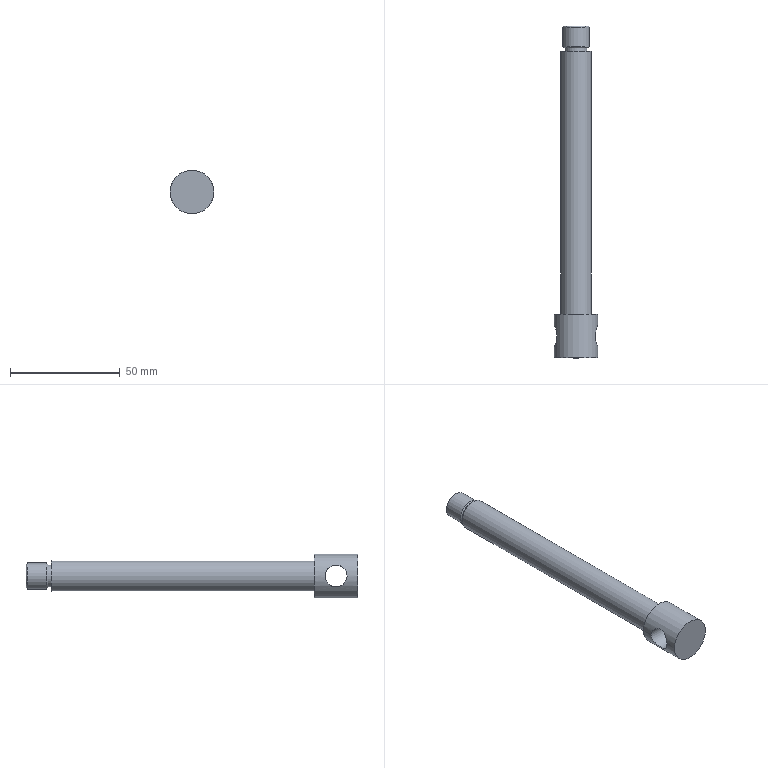Component | NX | SCREW_ROD | 1 solid | 12 faces | box 20 x 151.5 x 20 mm | volume 24476 mm3 | cylinder 5 | plane 5 | cone 2 | commonest cylinder face diameters 10 x2 20 x1 12 x1 14 x1
STEP:
#1=CARTESIAN_POINT('',(0.,0.,0.));
#2=DIRECTION('',(0.,0.,1.));
#3=DIRECTION('',(1.,0.,0.));
#4=AXIS2_PLACEMENT_3D('',#1,#2,#3);
#5=CARTESIAN_POINT('',(10.,-150.,-189.));
#6=VERTEX_POINT('',#5);
#7=CARTESIAN_POINT('',(0.,-150.,-189.));
#8=DIRECTION('',(0.,-1.,0.));
#9=DIRECTION('',(1.,0.,0.));
#10=AXIS2_PLACEMENT_3D('',#7,#8,#9);
#11=CIRCLE('',#10,10.);
#12=CARTESIAN_POINT('',(0.,-150.,-189.));
#13=DIRECTION('',(0.,1.,0.));
#14=DIRECTION('',(-1.,0.,0.));
#15=AXIS2_PLACEMENT_3D('',#12,#13,#14);
#16=CYLINDRICAL_SURFACE('',#15,10.);
#17=CARTESIAN_POINT('',(9.425,0.));
#18=DIRECTION('',(-1.,0.));
#19=VECTOR('',#18,1.);
#20=LINE('',#17,#19);
#21=(GEOMETRIC_REPRESENTATION_CONTEXT(2)PARAMETRIC_REPRESENTATION_CONTEXT()REPRESENTATION_CONTEXT('',''));
#22=DEFINITIONAL_REPRESENTATION('',(#20),#21);
#23=PCURVE('',#16,#22);
#24=CARTESIAN_POINT('',(0.,-150.,-189.));
#25=DIRECTION('',(0.,-1.,0.));
#26=DIRECTION('',(1.,0.,0.));
#27=AXIS2_PLACEMENT_3D('',#24,#25,#26);
#28=PLANE('',#27);
#29=CARTESIAN_POINT('',(0.,0.));
#30=DIRECTION('',(1.,0.));
#31=AXIS2_PLACEMENT_2D('',#29,#30);
#32=CIRCLE('',#31,10.);
#33=(GEOMETRIC_REPRESENTATION_CONTEXT(2)PARAMETRIC_REPRESENTATION_CONTEXT()REPRESENTATION_CONTEXT('',''));
#34=DEFINITIONAL_REPRESENTATION('',(#32),#33);
#35=PCURVE('',#28,#34);
#36=SURFACE_CURVE('',#11,(#23,#35),.PCURVE_S1.);
#37=EDGE_CURVE('',#6,#6,#36,.T.);
#38=ORIENTED_EDGE('',*,*,#37,.F.);
#39=CARTESIAN_POINT('',(10.,-145.,-189.));
#40=VERTEX_POINT('',#39);
#41=CARTESIAN_POINT('',(10.,-150.,-189.));
#42=CARTESIAN_POINT('',(10.,-145.,-189.));
#43=B_SPLINE_CURVE_WITH_KNOTS('',1,(#41,#42),.UNSPECIFIED.,.F.,.F.,(2,2),(0.,5.),.PIECEWISE_BEZIER_KNOTS.);
#44=CARTESIAN_POINT('',(9.425,0.));
#45=DIRECTION('',(0.,1.));
#46=VECTOR('',#45,1.);
#47=LINE('',#44,#46);
#48=(GEOMETRIC_REPRESENTATION_CONTEXT(2)PARAMETRIC_REPRESENTATION_CONTEXT()REPRESENTATION_CONTEXT('',''));
#49=DEFINITIONAL_REPRESENTATION('',(#47),#48);
#50=PCURVE('',#16,#49);
#51=CARTESIAN_POINT('',(3.142,0.));
#52=DIRECTION('',(0.,1.));
#53=VECTOR('',#52,1.);
#54=LINE('',#51,#53);
#55=(GEOMETRIC_REPRESENTATION_CONTEXT(2)PARAMETRIC_REPRESENTATION_CONTEXT()REPRESENTATION_CONTEXT('',''));
#56=DEFINITIONAL_REPRESENTATION('',(#54),#55);
#57=PCURVE('',#16,#56);
#58=SEAM_CURVE('',#43,(#50,#57),.PCURVE_S1.);
#59=EDGE_CURVE('',#6,#40,#58,.T.);
#60=ORIENTED_EDGE('',*,*,#59,.T.);
#61=CARTESIAN_POINT('',(10.,-135.,-189.));
#62=VERTEX_POINT('',#61);
#63=CARTESIAN_POINT('',(10.,-145.,-187.655));
#64=CARTESIAN_POINT('',(10.,-145.,-190.345));
#65=CARTESIAN_POINT('',(9.696,-144.44,-191.632));
#66=CARTESIAN_POINT('',(9.011,-142.627,-193.443));
#67=CARTESIAN_POINT('',(8.662,-141.341,-193.997));
#68=CARTESIAN_POINT('',(8.658,-138.682,-194.003));
#69=CARTESIAN_POINT('',(9.009,-137.38,-193.448));
#70=CARTESIAN_POINT('',(9.694,-135.563,-191.638));
#71=CARTESIAN_POINT('',(9.998,-135.004,-190.34));
#72=CARTESIAN_POINT('',(10.002,-134.996,-187.687));
#73=CARTESIAN_POINT('',(9.699,-135.553,-186.377));
#74=CARTESIAN_POINT('',(9.011,-137.371,-184.556));
#75=CARTESIAN_POINT('',(8.662,-138.664,-184.003));
#76=CARTESIAN_POINT('',(8.658,-141.312,-183.997));
#77=CARTESIAN_POINT('',(9.007,-142.615,-184.547));
#78=CARTESIAN_POINT('',(9.697,-144.445,-186.371));
#79=CARTESIAN_POINT('',(10.,-145.,-187.655));
#80=CARTESIAN_POINT('',(10.,-145.,-190.345));
#81=B_SPLINE_CURVE_WITH_KNOTS('',3,(#63,#64,#65,#66,#67,#68,#69,#70,#71,#72,#73,#74,#75,#76,#77,#78,#79,#80),.UNSPECIFIED.,.T.,.F.,(2,2,2,2,2,2,2,2,2,2,2),(-0.125,0.,0.125,0.25,0.375,0.5,0.625,0.75,0.875,1.,1.125),.UNSPECIFIED.);
#82=CARTESIAN_POINT('',(9.425,5.));
#83=CARTESIAN_POINT('',(9.449,5.));
#84=CARTESIAN_POINT('',(9.498,5.037));
#85=CARTESIAN_POINT('',(9.569,5.196));
#86=CARTESIAN_POINT('',(9.637,5.45));
#87=CARTESIAN_POINT('',(9.701,5.793));
#88=CARTESIAN_POINT('',(9.76,6.216));
#89=CARTESIAN_POINT('',(9.813,6.711));
#90=CARTESIAN_POINT('',(9.859,7.276));
#91=CARTESIAN_POINT('',(9.897,7.898));
#92=CARTESIAN_POINT('',(9.926,8.566));
#93=CARTESIAN_POINT('',(9.944,9.266));
#94=CARTESIAN_POINT('',(9.951,9.988));
#95=CARTESIAN_POINT('',(9.944,10.712));
#96=CARTESIAN_POINT('',(9.926,11.415));
#97=CARTESIAN_POINT('',(9.897,12.087));
#98=CARTESIAN_POINT('',(9.86,12.714));
#99=CARTESIAN_POINT('',(9.814,13.283));
#100=CARTESIAN_POINT('',(9.761,13.779));
#101=CARTESIAN_POINT('',(9.701,14.203));
#102=CARTESIAN_POINT('',(9.637,14.546));
#103=CARTESIAN_POINT('',(9.569,14.801));
#104=CARTESIAN_POINT('',(9.498,14.961));
#105=CARTESIAN_POINT('',(9.426,15.018));
#106=CARTESIAN_POINT('',(9.354,14.965));
#107=CARTESIAN_POINT('',(9.283,14.808));
#108=CARTESIAN_POINT('',(9.214,14.554));
#109=CARTESIAN_POINT('',(9.15,14.212));
#110=CARTESIAN_POINT('',(9.09,13.789));
#111=CARTESIAN_POINT('',(9.037,13.292));
#112=CARTESIAN_POINT('',(8.991,12.725));
#113=CARTESIAN_POINT('',(8.953,12.101));
#114=CARTESIAN_POINT('',(8.924,11.432));
#115=CARTESIAN_POINT('',(8.906,10.733));
#116=CARTESIAN_POINT('',(8.899,10.013));
#117=CARTESIAN_POINT('',(8.905,9.291));
#118=CARTESIAN_POINT('',(8.923,8.589));
#119=CARTESIAN_POINT('',(8.952,7.917));
#120=CARTESIAN_POINT('',(8.99,7.288));
#121=CARTESIAN_POINT('',(9.036,6.717));
#122=CARTESIAN_POINT('',(9.089,6.217));
#123=CARTESIAN_POINT('',(9.149,5.792));
#124=CARTESIAN_POINT('',(9.213,5.449));
#125=CARTESIAN_POINT('',(9.281,5.195));
#126=CARTESIAN_POINT('',(9.352,5.037));
#127=CARTESIAN_POINT('',(9.4,5.));
#128=CARTESIAN_POINT('',(9.425,5.));
#129=B_SPLINE_CURVE_WITH_KNOTS('',3,(#82,#83,#84,#85,#86,#87,#88,#89,#90,#91,#92,#93,#94,#95,#96,#97,#98,#99,#100,#101,#102,#103,#104,#105,#106,#107,#108,#109,#110,#111,#112,#113,#114,#115,#116,#117,#118,#119,#120,#121,#122,#123,#124,#125,#126,#127,#128),.UNSPECIFIED.,.T.,.F.,(4,1,1,1,1,1,1,1,1,1,1,1,1,1,1,1,1,1,1,1,1,1,1,1,1,1,1,1,1,1,1,1,1,1,1,1,1,1,1,1,1,1,1,1,4),(0.,0.02273,0.04545,0.06818,0.09091,0.1136,0.1364,0.1591,0.1818,0.2045,0.2273,0.25,0.2727,0.2955,0.3182,0.3409,0.3636,0.3864,0.4091,0.4318,0.4545,0.4773,0.5,0.5227,0.5455,0.5682,0.5909,0.6136,0.6364,0.6591,0.6818,0.7045,0.7273,0.75,0.7727,0.7955,0.8182,0.8409,0.8636,0.8864,0.9091,0.9318,0.9545,0.9773,1.),.QUASI_UNIFORM_KNOTS.);
#130=(GEOMETRIC_REPRESENTATION_CONTEXT(2)PARAMETRIC_REPRESENTATION_CONTEXT()REPRESENTATION_CONTEXT('',''));
#131=DEFINITIONAL_REPRESENTATION('',(#129),#130);
#132=PCURVE('',#16,#131);
#133=CARTESIAN_POINT('',(20.,-140.,-189.));
#134=DIRECTION('',(-1.,0.,0.));
#135=DIRECTION('',(0.,-1.,0.));
#136=AXIS2_PLACEMENT_3D('',#133,#134,#135);
#137=CYLINDRICAL_SURFACE('',#136,5.);
#138=CARTESIAN_POINT('',(3.142,10.));
#139=CARTESIAN_POINT('',(3.093,10.));
#140=CARTESIAN_POINT('',(2.997,10.02));
#141=CARTESIAN_POINT('',(2.853,10.101));
#142=CARTESIAN_POINT('',(2.709,10.223));
#143=CARTESIAN_POINT('',(2.566,10.377));
#144=CARTESIAN_POINT('',(2.425,10.553));
#145=CARTESIAN_POINT('',(2.285,10.742));
#146=CARTESIAN_POINT('',(2.144,10.926));
#147=CARTESIAN_POINT('',(2.002,11.091));
#148=CARTESIAN_POINT('',(1.859,11.225));
#149=CARTESIAN_POINT('',(1.716,11.316));
#150=CARTESIAN_POINT('',(1.572,11.351));
#151=CARTESIAN_POINT('',(1.428,11.317));
#152=CARTESIAN_POINT('',(1.284,11.226));
#153=CARTESIAN_POINT('',(1.141,11.092));
#154=CARTESIAN_POINT('',(0.9984,10.926));
#155=CARTESIAN_POINT('',(0.8566,10.742));
#156=CARTESIAN_POINT('',(0.716,10.552));
#157=CARTESIAN_POINT('',(0.5747,10.376));
#158=CARTESIAN_POINT('',(0.4326,10.222));
#159=CARTESIAN_POINT('',(0.2897,10.101));
#160=CARTESIAN_POINT('',(0.1458,10.02));
#161=CARTESIAN_POINT('',(0.04883,10.));
#162=CARTESIAN_POINT('',(0.,10.));
#163=B_SPLINE_CURVE_WITH_KNOTS('',3,(#138,#139,#140,#141,#142,#143,#144,#145,#146,#147,#148,#149,#150,#151,#152,#153,#154,#155,#156,#157,#158,#159,#160,#161,#162),.UNSPECIFIED.,.F.,.F.,(4,1,1,1,1,1,1,1,1,1,1,1,1,1,1,1,1,1,1,1,1,1,4),(0.5004,0.5231,0.5459,0.5686,0.5913,0.614,0.6367,0.6594,0.6821,0.7048,0.7275,0.7502,0.7729,0.7956,0.8183,0.841,0.8638,0.8865,0.9092,0.9319,0.9546,0.9773,1.),.QUASI_UNIFORM_KNOTS.);
#164=(GEOMETRIC_REPRESENTATION_CONTEXT(2)PARAMETRIC_REPRESENTATION_CONTEXT()REPRESENTATION_CONTEXT('',''));
#165=DEFINITIONAL_REPRESENTATION('',(#163),#164);
#166=PCURVE('',#137,#165);
#167=SURFACE_CURVE('',#81,(#132,#166),.PCURVE_S1.);
#168=EDGE_CURVE('',#62,#40,#167,.T.);
#169=ORIENTED_EDGE('',*,*,#168,.F.);
#170=CARTESIAN_POINT('',(10.,-130.,-189.));
#171=VERTEX_POINT('',#170);
#172=CARTESIAN_POINT('',(10.,-135.,-189.));
#173=CARTESIAN_POINT('',(10.,-130.,-189.));
#174=B_SPLINE_CURVE_WITH_KNOTS('',1,(#172,#173),.UNSPECIFIED.,.F.,.F.,(2,2),(15.,20.),.PIECEWISE_BEZIER_KNOTS.);
#175=CARTESIAN_POINT('',(9.425,0.));
#176=DIRECTION('',(0.,1.));
#177=VECTOR('',#176,1.);
#178=LINE('',#175,#177);
#179=(GEOMETRIC_REPRESENTATION_CONTEXT(2)PARAMETRIC_REPRESENTATION_CONTEXT()REPRESENTATION_CONTEXT('',''));
#180=DEFINITIONAL_REPRESENTATION('',(#178),#179);
#181=PCURVE('',#16,#180);
#182=CARTESIAN_POINT('',(3.142,0.));
#183=DIRECTION('',(0.,1.));
#184=VECTOR('',#183,1.);
#185=LINE('',#182,#184);
#186=(GEOMETRIC_REPRESENTATION_CONTEXT(2)PARAMETRIC_REPRESENTATION_CONTEXT()REPRESENTATION_CONTEXT('',''));
#187=DEFINITIONAL_REPRESENTATION('',(#185),#186);
#188=PCURVE('',#16,#187);
#189=SEAM_CURVE('',#174,(#181,#188),.PCURVE_S1.);
#190=EDGE_CURVE('',#62,#171,#189,.T.);
#191=ORIENTED_EDGE('',*,*,#190,.T.);
#192=CARTESIAN_POINT('',(0.,-130.,-189.));
#193=DIRECTION('',(0.,-1.,0.));
#194=DIRECTION('',(1.,0.,0.));
#195=AXIS2_PLACEMENT_3D('',#192,#193,#194);
#196=CIRCLE('',#195,10.);
#197=CARTESIAN_POINT('',(9.425,20.));
#198=DIRECTION('',(-1.,0.));
#199=VECTOR('',#198,1.);
#200=LINE('',#197,#199);
#201=(GEOMETRIC_REPRESENTATION_CONTEXT(2)PARAMETRIC_REPRESENTATION_CONTEXT()REPRESENTATION_CONTEXT('',''));
#202=DEFINITIONAL_REPRESENTATION('',(#200),#201);
#203=PCURVE('',#16,#202);
#204=CARTESIAN_POINT('',(0.,-130.,-189.));
#205=DIRECTION('',(0.,-1.,0.));
#206=DIRECTION('',(1.,0.,0.));
#207=AXIS2_PLACEMENT_3D('',#204,#205,#206);
#208=PLANE('',#207);
#209=CARTESIAN_POINT('',(0.,0.));
#210=DIRECTION('',(1.,0.));
#211=AXIS2_PLACEMENT_2D('',#209,#210);
#212=CIRCLE('',#211,10.);
#213=(GEOMETRIC_REPRESENTATION_CONTEXT(2)PARAMETRIC_REPRESENTATION_CONTEXT()REPRESENTATION_CONTEXT('',''));
#214=DEFINITIONAL_REPRESENTATION('',(#212),#213);
#215=PCURVE('',#208,#214);
#216=SURFACE_CURVE('',#196,(#203,#215),.PCURVE_S1.);
#217=EDGE_CURVE('',#171,#171,#216,.T.);
#218=ORIENTED_EDGE('',*,*,#217,.T.);
#219=ORIENTED_EDGE('',*,*,#190,.F.);
#220=CARTESIAN_POINT('',(10.,-145.,-187.655));
#221=CARTESIAN_POINT('',(10.,-145.,-190.345));
#222=CARTESIAN_POINT('',(9.696,-144.44,-191.632));
#223=CARTESIAN_POINT('',(9.011,-142.627,-193.443));
#224=CARTESIAN_POINT('',(8.662,-141.341,-193.997));
#225=CARTESIAN_POINT('',(8.658,-138.682,-194.003));
#226=CARTESIAN_POINT('',(9.009,-137.38,-193.448));
#227=CARTESIAN_POINT('',(9.694,-135.563,-191.638));
#228=CARTESIAN_POINT('',(9.998,-135.004,-190.34));
#229=CARTESIAN_POINT('',(10.002,-134.996,-187.687));
#230=CARTESIAN_POINT('',(9.699,-135.553,-186.377));
#231=CARTESIAN_POINT('',(9.011,-137.371,-184.556));
#232=CARTESIAN_POINT('',(8.662,-138.664,-184.003));
#233=CARTESIAN_POINT('',(8.658,-141.312,-183.997));
#234=CARTESIAN_POINT('',(9.007,-142.615,-184.547));
#235=CARTESIAN_POINT('',(9.697,-144.445,-186.371));
#236=CARTESIAN_POINT('',(10.,-145.,-187.655));
#237=CARTESIAN_POINT('',(10.,-145.,-190.345));
#238=B_SPLINE_CURVE_WITH_KNOTS('',3,(#220,#221,#222,#223,#224,#225,#226,#227,#228,#229,#230,#231,#232,#233,#234,#235,#236,#237),.UNSPECIFIED.,.T.,.F.,(2,2,2,2,2,2,2,2,2,2,2),(-0.125,0.,0.125,0.25,0.375,0.5,0.625,0.75,0.875,1.,1.125),.UNSPECIFIED.);
#239=CARTESIAN_POINT('',(3.142,5.));
#240=CARTESIAN_POINT('',(3.166,5.));
#241=CARTESIAN_POINT('',(3.215,5.037));
#242=CARTESIAN_POINT('',(3.285,5.196));
#243=CARTESIAN_POINT('',(3.354,5.45));
#244=CARTESIAN_POINT('',(3.418,5.793));
#245=CARTESIAN_POINT('',(3.477,6.216));
#246=CARTESIAN_POINT('',(3.53,6.711));
#247=CARTESIAN_POINT('',(3.576,7.276));
#248=CARTESIAN_POINT('',(3.614,7.898));
#249=CARTESIAN_POINT('',(3.642,8.566));
#250=CARTESIAN_POINT('',(3.661,9.266));
#251=CARTESIAN_POINT('',(3.667,9.988));
#252=CARTESIAN_POINT('',(3.661,10.712));
#253=CARTESIAN_POINT('',(3.643,11.415));
#254=CARTESIAN_POINT('',(3.614,12.087));
#255=CARTESIAN_POINT('',(3.576,12.714));
#256=CARTESIAN_POINT('',(3.53,13.283));
#257=CARTESIAN_POINT('',(3.478,13.779));
#258=CARTESIAN_POINT('',(3.418,14.203));
#259=CARTESIAN_POINT('',(3.354,14.546));
#260=CARTESIAN_POINT('',(3.286,14.801));
#261=CARTESIAN_POINT('',(3.215,14.961));
#262=CARTESIAN_POINT('',(3.143,15.018));
#263=CARTESIAN_POINT('',(3.071,14.965));
#264=CARTESIAN_POINT('',(3.,14.808));
#265=CARTESIAN_POINT('',(2.931,14.554));
#266=CARTESIAN_POINT('',(2.866,14.212));
#267=CARTESIAN_POINT('',(2.807,13.789));
#268=CARTESIAN_POINT('',(2.754,13.292));
#269=CARTESIAN_POINT('',(2.707,12.725));
#270=CARTESIAN_POINT('',(2.67,12.101));
#271=CARTESIAN_POINT('',(2.641,11.432));
#272=CARTESIAN_POINT('',(2.622,10.733));
#273=CARTESIAN_POINT('',(2.616,10.013));
#274=CARTESIAN_POINT('',(2.622,9.291));
#275=CARTESIAN_POINT('',(2.64,8.589));
#276=CARTESIAN_POINT('',(2.669,7.917));
#277=CARTESIAN_POINT('',(2.707,7.288));
#278=CARTESIAN_POINT('',(2.753,6.717));
#279=CARTESIAN_POINT('',(2.806,6.217));
#280=CARTESIAN_POINT('',(2.865,5.792));
#281=CARTESIAN_POINT('',(2.93,5.449));
#282=CARTESIAN_POINT('',(2.998,5.195));
#283=CARTESIAN_POINT('',(3.069,5.037));
#284=CARTESIAN_POINT('',(3.117,5.));
#285=CARTESIAN_POINT('',(3.142,5.));
#286=B_SPLINE_CURVE_WITH_KNOTS('',3,(#239,#240,#241,#242,#243,#244,#245,#246,#247,#248,#249,#250,#251,#252,#253,#254,#255,#256,#257,#258,#259,#260,#261,#262,#263,#264,#265,#266,#267,#268,#269,#270,#271,#272,#273,#274,#275,#276,#277,#278,#279,#280,#281,#282,#283,#284,#285),.UNSPECIFIED.,.T.,.F.,(4,1,1,1,1,1,1,1,1,1,1,1,1,1,1,1,1,1,1,1,1,1,1,1,1,1,1,1,1,1,1,1,1,1,1,1,1,1,1,1,1,1,1,1,4),(0.,0.02273,0.04545,0.06818,0.09091,0.1136,0.1364,0.1591,0.1818,0.2045,0.2273,0.25,0.2727,0.2955,0.3182,0.3409,0.3636,0.3864,0.4091,0.4318,0.4545,0.4773,0.5,0.5227,0.5455,0.5682,0.5909,0.6136,0.6364,0.6591,0.6818,0.7045,0.7273,0.75,0.7727,0.7955,0.8182,0.8409,0.8636,0.8864,0.9091,0.9318,0.9545,0.9773,1.),.QUASI_UNIFORM_KNOTS.);
#287=(GEOMETRIC_REPRESENTATION_CONTEXT(2)PARAMETRIC_REPRESENTATION_CONTEXT()REPRESENTATION_CONTEXT('',''));
#288=DEFINITIONAL_REPRESENTATION('',(#286),#287);
#289=PCURVE('',#16,#288);
#290=CARTESIAN_POINT('',(6.283,10.));
#291=CARTESIAN_POINT('',(6.234,10.));
#292=CARTESIAN_POINT('',(6.137,10.02));
#293=CARTESIAN_POINT('',(5.993,10.101));
#294=CARTESIAN_POINT('',(5.85,10.223));
#295=CARTESIAN_POINT('',(5.708,10.377));
#296=CARTESIAN_POINT('',(5.567,10.553));
#297=CARTESIAN_POINT('',(5.427,10.742));
#298=CARTESIAN_POINT('',(5.286,10.925));
#299=CARTESIAN_POINT('',(5.144,11.09));
#300=CARTESIAN_POINT('',(5.001,11.225));
#301=CARTESIAN_POINT('',(4.858,11.316));
#302=CARTESIAN_POINT('',(4.713,11.351));
#303=CARTESIAN_POINT('',(4.568,11.317));
#304=CARTESIAN_POINT('',(4.424,11.225));
#305=CARTESIAN_POINT('',(4.281,11.09));
#306=CARTESIAN_POINT('',(4.138,10.924));
#307=CARTESIAN_POINT('',(3.997,10.74));
#308=CARTESIAN_POINT('',(3.857,10.551));
#309=CARTESIAN_POINT('',(3.716,10.376));
#310=CARTESIAN_POINT('',(3.573,10.222));
#311=CARTESIAN_POINT('',(3.43,10.101));
#312=CARTESIAN_POINT('',(3.286,10.02));
#313=CARTESIAN_POINT('',(3.19,10.));
#314=CARTESIAN_POINT('',(3.142,10.));
#315=B_SPLINE_CURVE_WITH_KNOTS('',3,(#290,#291,#292,#293,#294,#295,#296,#297,#298,#299,#300,#301,#302,#303,#304,#305,#306,#307,#308,#309,#310,#311,#312,#313,#314),.UNSPECIFIED.,.F.,.F.,(4,1,1,1,1,1,1,1,1,1,1,1,1,1,1,1,1,1,1,1,1,1,4),(0.,0.02275,0.04549,0.06824,0.09099,0.1137,0.1365,0.1592,0.182,0.2047,0.2275,0.2502,0.273,0.2957,0.3185,0.3412,0.364,0.3867,0.4094,0.4322,0.4549,0.4777,0.5004),.QUASI_UNIFORM_KNOTS.);
#316=(GEOMETRIC_REPRESENTATION_CONTEXT(2)PARAMETRIC_REPRESENTATION_CONTEXT()REPRESENTATION_CONTEXT('',''));
#317=DEFINITIONAL_REPRESENTATION('',(#315),#316);
#318=PCURVE('',#137,#317);
#319=SURFACE_CURVE('',#238,(#289,#318),.PCURVE_S1.);
#320=EDGE_CURVE('',#40,#62,#319,.T.);
#321=ORIENTED_EDGE('',*,*,#320,.F.);
#322=ORIENTED_EDGE('',*,*,#59,.F.);
#323=EDGE_LOOP('',(#38,#60,#169,#191,#218,#219,#321,#322));
#324=FACE_BOUND('',#323,.T.);
#325=CARTESIAN_POINT('',(-10.,-145.,-189.));
#326=VERTEX_POINT('',#325);
#327=CARTESIAN_POINT('',(-10.,-145.,-190.345));
#328=CARTESIAN_POINT('',(-10.,-145.,-187.655));
#329=CARTESIAN_POINT('',(-9.696,-144.44,-186.368));
#330=CARTESIAN_POINT('',(-9.011,-142.627,-184.557));
#331=CARTESIAN_POINT('',(-8.662,-141.341,-184.003));
#332=CARTESIAN_POINT('',(-8.658,-138.682,-183.997));
#333=CARTESIAN_POINT('',(-9.009,-137.38,-184.552));
#334=CARTESIAN_POINT('',(-9.694,-135.563,-186.362));
#335=CARTESIAN_POINT('',(-9.998,-135.004,-187.66));
#336=CARTESIAN_POINT('',(-10.002,-134.996,-190.313));
#337=CARTESIAN_POINT('',(-9.699,-135.553,-191.623));
#338=CARTESIAN_POINT('',(-9.011,-137.371,-193.444));
#339=CARTESIAN_POINT('',(-8.662,-138.664,-193.997));
#340=CARTESIAN_POINT('',(-8.658,-141.312,-194.003));
#341=CARTESIAN_POINT('',(-9.007,-142.615,-193.453));
#342=CARTESIAN_POINT('',(-9.697,-144.445,-191.629));
#343=CARTESIAN_POINT('',(-10.,-145.,-190.345));
#344=CARTESIAN_POINT('',(-10.,-145.,-187.655));
#345=B_SPLINE_CURVE_WITH_KNOTS('',3,(#327,#328,#329,#330,#331,#332,#333,#334,#335,#336,#337,#338,#339,#340,#341,#342,#343,#344),.UNSPECIFIED.,.T.,.F.,(2,2,2,2,2,2,2,2,2,2,2),(-0.125,0.,0.125,0.25,0.375,0.5,0.625,0.75,0.875,1.,1.125),.UNSPECIFIED.);
#346=CARTESIAN_POINT('',(6.283,5.));
#347=CARTESIAN_POINT('',(6.308,5.));
#348=CARTESIAN_POINT('',(6.356,5.037));
#349=CARTESIAN_POINT('',(6.427,5.196));
#350=CARTESIAN_POINT('',(6.495,5.45));
#351=CARTESIAN_POINT('',(6.559,5.793));
#352=CARTESIAN_POINT('',(6.619,6.216));
#353=CARTESIAN_POINT('',(6.671,6.711));
#354=CARTESIAN_POINT('',(6.717,7.276));
#355=CARTESIAN_POINT('',(6.755,7.898));
#356=CARTESIAN_POINT('',(6.784,8.566));
#357=CARTESIAN_POINT('',(6.802,9.266));
#358=CARTESIAN_POINT('',(6.809,9.988));
#359=CARTESIAN_POINT('',(6.803,10.712));
#360=CARTESIAN_POINT('',(6.784,11.415));
#361=CARTESIAN_POINT('',(6.756,12.087));
#362=CARTESIAN_POINT('',(6.718,12.714));
#363=CARTESIAN_POINT('',(6.672,13.283));
#364=CARTESIAN_POINT('',(6.619,13.779));
#365=CARTESIAN_POINT('',(6.56,14.203));
#366=CARTESIAN_POINT('',(6.496,14.546));
#367=CARTESIAN_POINT('',(6.427,14.801));
#368=CARTESIAN_POINT('',(6.357,14.961));
#369=CARTESIAN_POINT('',(6.285,15.018));
#370=CARTESIAN_POINT('',(6.212,14.965));
#371=CARTESIAN_POINT('',(6.141,14.808));
#372=CARTESIAN_POINT('',(6.073,14.554));
#373=CARTESIAN_POINT('',(6.008,14.212));
#374=CARTESIAN_POINT('',(5.948,13.789));
#375=CARTESIAN_POINT('',(5.895,13.292));
#376=CARTESIAN_POINT('',(5.849,12.725));
#377=CARTESIAN_POINT('',(5.811,12.101));
#378=CARTESIAN_POINT('',(5.782,11.432));
#379=CARTESIAN_POINT('',(5.764,10.733));
#380=CARTESIAN_POINT('',(5.757,10.013));
#381=CARTESIAN_POINT('',(5.764,9.291));
#382=CARTESIAN_POINT('',(5.782,8.589));
#383=CARTESIAN_POINT('',(5.81,7.917));
#384=CARTESIAN_POINT('',(5.848,7.288));
#385=CARTESIAN_POINT('',(5.894,6.717));
#386=CARTESIAN_POINT('',(5.948,6.217));
#387=CARTESIAN_POINT('',(6.007,5.792));
#388=CARTESIAN_POINT('',(6.071,5.449));
#389=CARTESIAN_POINT('',(6.139,5.195));
#390=CARTESIAN_POINT('',(6.21,5.037));
#391=CARTESIAN_POINT('',(6.259,5.));
#392=CARTESIAN_POINT('',(6.283,5.));
#393=B_SPLINE_CURVE_WITH_KNOTS('',3,(#346,#347,#348,#349,#350,#351,#352,#353,#354,#355,#356,#357,#358,#359,#360,#361,#362,#363,#364,#365,#366,#367,#368,#369,#370,#371,#372,#373,#374,#375,#376,#377,#378,#379,#380,#381,#382,#383,#384,#385,#386,#387,#388,#389,#390,#391,#392),.UNSPECIFIED.,.T.,.F.,(4,1,1,1,1,1,1,1,1,1,1,1,1,1,1,1,1,1,1,1,1,1,1,1,1,1,1,1,1,1,1,1,1,1,1,1,1,1,1,1,1,1,1,1,4),(0.,0.02273,0.04545,0.06818,0.09091,0.1136,0.1364,0.1591,0.1818,0.2045,0.2273,0.25,0.2727,0.2955,0.3182,0.3409,0.3636,0.3864,0.4091,0.4318,0.4545,0.4773,0.5,0.5227,0.5455,0.5682,0.5909,0.6136,0.6364,0.6591,0.6818,0.7045,0.7273,0.75,0.7727,0.7955,0.8182,0.8409,0.8636,0.8864,0.9091,0.9318,0.9545,0.9773,1.),.QUASI_UNIFORM_KNOTS.);
#394=(GEOMETRIC_REPRESENTATION_CONTEXT(2)PARAMETRIC_REPRESENTATION_CONTEXT()REPRESENTATION_CONTEXT('',''));
#395=DEFINITIONAL_REPRESENTATION('',(#393),#394);
#396=PCURVE('',#16,#395);
#397=CARTESIAN_POINT('',(0.,30.));
#398=CARTESIAN_POINT('',(0.04886,30.));
#399=CARTESIAN_POINT('',(0.146,29.98));
#400=CARTESIAN_POINT('',(0.2901,29.899));
#401=CARTESIAN_POINT('',(0.4332,29.777));
#402=CARTESIAN_POINT('',(0.5752,29.623));
#403=CARTESIAN_POINT('',(0.7161,29.448));
#404=CARTESIAN_POINT('',(0.8557,29.259));
#405=CARTESIAN_POINT('',(0.9964,29.076));
#406=CARTESIAN_POINT('',(1.138,28.911));
#407=CARTESIAN_POINT('',(1.281,28.776));
#408=CARTESIAN_POINT('',(1.424,28.684));
#409=CARTESIAN_POINT('',(1.568,28.649));
#410=CARTESIAN_POINT('',(1.713,28.683));
#411=CARTESIAN_POINT('',(1.857,28.773));
#412=CARTESIAN_POINT('',(2.,28.908));
#413=CARTESIAN_POINT('',(2.143,29.074));
#414=CARTESIAN_POINT('',(2.284,29.257));
#415=CARTESIAN_POINT('',(2.424,29.446));
#416=CARTESIAN_POINT('',(2.565,29.621));
#417=CARTESIAN_POINT('',(2.708,29.775));
#418=CARTESIAN_POINT('',(2.851,29.898));
#419=CARTESIAN_POINT('',(2.994,29.979));
#420=CARTESIAN_POINT('',(3.139,30.01));
#421=CARTESIAN_POINT('',(3.283,29.981));
#422=CARTESIAN_POINT('',(3.428,29.901));
#423=CARTESIAN_POINT('',(3.571,29.779));
#424=CARTESIAN_POINT('',(3.714,29.626));
#425=CARTESIAN_POINT('',(3.856,29.45));
#426=CARTESIAN_POINT('',(3.996,29.26));
#427=CARTESIAN_POINT('',(4.138,29.077));
#428=CARTESIAN_POINT('',(4.28,28.911));
#429=CARTESIAN_POINT('',(4.423,28.776));
#430=CARTESIAN_POINT('',(4.566,28.684));
#431=CARTESIAN_POINT('',(4.71,28.649));
#432=CARTESIAN_POINT('',(4.854,28.682));
#433=CARTESIAN_POINT('',(4.998,28.773));
#434=CARTESIAN_POINT('',(5.141,28.907));
#435=CARTESIAN_POINT('',(5.284,29.073));
#436=CARTESIAN_POINT('',(5.426,29.257));
#437=CARTESIAN_POINT('',(5.567,29.447));
#438=CARTESIAN_POINT('',(5.708,29.623));
#439=CARTESIAN_POINT('',(5.85,29.777));
#440=CARTESIAN_POINT('',(5.993,29.899));
#441=CARTESIAN_POINT('',(6.137,29.98));
#442=CARTESIAN_POINT('',(6.234,30.));
#443=CARTESIAN_POINT('',(6.283,30.));
#444=B_SPLINE_CURVE_WITH_KNOTS('',3,(#397,#398,#399,#400,#401,#402,#403,#404,#405,#406,#407,#408,#409,#410,#411,#412,#413,#414,#415,#416,#417,#418,#419,#420,#421,#422,#423,#424,#425,#426,#427,#428,#429,#430,#431,#432,#433,#434,#435,#436,#437,#438,#439,#440,#441,#442,#443),.UNSPECIFIED.,.F.,.F.,(4,1,1,1,1,1,1,1,1,1,1,1,1,1,1,1,1,1,1,1,1,1,1,1,1,1,1,1,1,1,1,1,1,1,1,1,1,1,1,1,1,1,1,1,4),(0.,0.02273,0.04545,0.06818,0.09091,0.1136,0.1364,0.1591,0.1818,0.2045,0.2273,0.25,0.2727,0.2955,0.3182,0.3409,0.3636,0.3864,0.4091,0.4318,0.4545,0.4773,0.5,0.5227,0.5455,0.5682,0.5909,0.6136,0.6364,0.6591,0.6818,0.7045,0.7273,0.75,0.7727,0.7955,0.8182,0.8409,0.8636,0.8864,0.9091,0.9318,0.9545,0.9773,1.),.QUASI_UNIFORM_KNOTS.);
#445=(GEOMETRIC_REPRESENTATION_CONTEXT(2)PARAMETRIC_REPRESENTATION_CONTEXT()REPRESENTATION_CONTEXT('',''));
#446=DEFINITIONAL_REPRESENTATION('',(#444),#445);
#447=PCURVE('',#137,#446);
#448=SURFACE_CURVE('',#345,(#396,#447),.PCURVE_S1.);
#449=EDGE_CURVE('',#326,#326,#448,.T.);
#450=ORIENTED_EDGE('',*,*,#449,.F.);
#451=EDGE_LOOP('',(#450));
#452=FACE_BOUND('',#451,.T.);
#453=ADVANCED_FACE('',(#324,#452),#16,.T.);
#454=CARTESIAN_POINT('',(6.,1.,-189.));
#455=VERTEX_POINT('',#454);
#456=CARTESIAN_POINT('',(0.,1.,-189.));
#457=DIRECTION('',(0.,-1.,0.));
#458=DIRECTION('',(1.,0.,0.));
#459=AXIS2_PLACEMENT_3D('',#456,#457,#458);
#460=CIRCLE('',#459,6.);
#461=CARTESIAN_POINT('',(0.,-8.5,-189.));
#462=DIRECTION('',(0.,1.,0.));
#463=DIRECTION('',(-1.,0.,0.));
#464=AXIS2_PLACEMENT_3D('',#461,#462,#463);
#465=CYLINDRICAL_SURFACE('',#464,6.);
#466=CARTESIAN_POINT('',(9.425,9.5));
#467=DIRECTION('',(-1.,0.));
#468=VECTOR('',#467,1.);
#469=LINE('',#466,#468);
#470=(GEOMETRIC_REPRESENTATION_CONTEXT(2)PARAMETRIC_REPRESENTATION_CONTEXT()REPRESENTATION_CONTEXT('',''));
#471=DEFINITIONAL_REPRESENTATION('',(#469),#470);
#472=PCURVE('',#465,#471);
#473=CARTESIAN_POINT('',(0.,1.,-189.));
#474=DIRECTION('',(0.,-1.,0.));
#475=DIRECTION('',(1.,0.,0.));
#476=AXIS2_PLACEMENT_3D('',#473,#474,#475);
#477=CONICAL_SURFACE('',#476,6.,0.7854);
#478=CARTESIAN_POINT('',(0.,0.));
#479=DIRECTION('',(1.,0.));
#480=VECTOR('',#479,1.);
#481=LINE('',#478,#480);
#482=(GEOMETRIC_REPRESENTATION_CONTEXT(2)PARAMETRIC_REPRESENTATION_CONTEXT()REPRESENTATION_CONTEXT('',''));
#483=DEFINITIONAL_REPRESENTATION('',(#481),#482);
#484=PCURVE('',#477,#483);
#485=SURFACE_CURVE('',#460,(#472,#484),.PCURVE_S1.);
#486=EDGE_CURVE('',#455,#455,#485,.T.);
#487=ORIENTED_EDGE('',*,*,#486,.T.);
#488=CARTESIAN_POINT('',(6.,-8.,-189.));
#489=VERTEX_POINT('',#488);
#490=CARTESIAN_POINT('',(6.,-8.,-189.));
#491=CARTESIAN_POINT('',(6.,1.,-189.));
#492=B_SPLINE_CURVE_WITH_KNOTS('',1,(#490,#491),.UNSPECIFIED.,.F.,.F.,(2,2),(0.5,9.5),.PIECEWISE_BEZIER_KNOTS.);
#493=CARTESIAN_POINT('',(3.142,0.));
#494=DIRECTION('',(0.,1.));
#495=VECTOR('',#494,1.);
#496=LINE('',#493,#495);
#497=(GEOMETRIC_REPRESENTATION_CONTEXT(2)PARAMETRIC_REPRESENTATION_CONTEXT()REPRESENTATION_CONTEXT('',''));
#498=DEFINITIONAL_REPRESENTATION('',(#496),#497);
#499=PCURVE('',#465,#498);
#500=CARTESIAN_POINT('',(9.425,0.));
#501=DIRECTION('',(0.,1.));
#502=VECTOR('',#501,1.);
#503=LINE('',#500,#502);
#504=(GEOMETRIC_REPRESENTATION_CONTEXT(2)PARAMETRIC_REPRESENTATION_CONTEXT()REPRESENTATION_CONTEXT('',''));
#505=DEFINITIONAL_REPRESENTATION('',(#503),#504);
#506=PCURVE('',#465,#505);
#507=SEAM_CURVE('',#492,(#499,#506),.PCURVE_S1.);
#508=EDGE_CURVE('',#489,#455,#507,.T.);
#509=ORIENTED_EDGE('',*,*,#508,.F.);
#510=CARTESIAN_POINT('',(0.,-8.,-189.));
#511=DIRECTION('',(0.,1.,0.));
#512=DIRECTION('',(1.,0.,0.));
#513=AXIS2_PLACEMENT_3D('',#510,#511,#512);
#514=CIRCLE('',#513,6.);
#515=CARTESIAN_POINT('',(3.142,0.5));
#516=DIRECTION('',(1.,0.));
#517=VECTOR('',#516,1.);
#518=LINE('',#515,#517);
#519=(GEOMETRIC_REPRESENTATION_CONTEXT(2)PARAMETRIC_REPRESENTATION_CONTEXT()REPRESENTATION_CONTEXT('',''));
#520=DEFINITIONAL_REPRESENTATION('',(#518),#519);
#521=PCURVE('',#465,#520);
#522=CARTESIAN_POINT('',(0.,-8.5,-189.));
#523=DIRECTION('',(0.,1.,0.));
#524=DIRECTION('',(-1.,0.,0.));
#525=AXIS2_PLACEMENT_3D('',#522,#523,#524);
#526=CONICAL_SURFACE('',#525,5.5,0.7854);
#527=CARTESIAN_POINT('',(3.142,0.5));
#528=DIRECTION('',(1.,0.));
#529=VECTOR('',#528,1.);
#530=LINE('',#527,#529);
#531=(GEOMETRIC_REPRESENTATION_CONTEXT(2)PARAMETRIC_REPRESENTATION_CONTEXT()REPRESENTATION_CONTEXT('',''));
#532=DEFINITIONAL_REPRESENTATION('',(#530),#531);
#533=PCURVE('',#526,#532);
#534=SURFACE_CURVE('',#514,(#521,#533),.PCURVE_S1.);
#535=EDGE_CURVE('',#489,#489,#534,.T.);
#536=ORIENTED_EDGE('',*,*,#535,.T.);
#537=ORIENTED_EDGE('',*,*,#508,.T.);
#538=EDGE_LOOP('',(#487,#509,#536,#537));
#539=FACE_BOUND('',#538,.T.);
#540=ADVANCED_FACE('',(#539),#465,.T.);
#541=CARTESIAN_POINT('',(5.5,-8.5,-189.));
#542=VERTEX_POINT('',#541);
#543=CARTESIAN_POINT('',(0.,-8.5,-189.));
#544=DIRECTION('',(0.,-1.,0.));
#545=DIRECTION('',(1.,0.,0.));
#546=AXIS2_PLACEMENT_3D('',#543,#544,#545);
#547=CIRCLE('',#546,5.5);
#548=CARTESIAN_POINT('',(0.,-8.5,-189.));
#549=DIRECTION('',(0.,-1.,0.));
#550=DIRECTION('',(1.,0.,0.));
#551=AXIS2_PLACEMENT_3D('',#548,#549,#550);
#552=PLANE('',#551);
#553=CARTESIAN_POINT('',(0.,0.));
#554=DIRECTION('',(1.,0.));
#555=AXIS2_PLACEMENT_2D('',#553,#554);
#556=CIRCLE('',#555,5.5);
#557=(GEOMETRIC_REPRESENTATION_CONTEXT(2)PARAMETRIC_REPRESENTATION_CONTEXT()REPRESENTATION_CONTEXT('',''));
#558=DEFINITIONAL_REPRESENTATION('',(#556),#557);
#559=PCURVE('',#552,#558);
#560=CARTESIAN_POINT('',(9.425,0.));
#561=DIRECTION('',(-1.,0.));
#562=VECTOR('',#561,1.);
#563=LINE('',#560,#562);
#564=(GEOMETRIC_REPRESENTATION_CONTEXT(2)PARAMETRIC_REPRESENTATION_CONTEXT()REPRESENTATION_CONTEXT('',''));
#565=DEFINITIONAL_REPRESENTATION('',(#563),#564);
#566=PCURVE('',#526,#565);
#567=SURFACE_CURVE('',#547,(#559,#566),.PCURVE_S1.);
#568=EDGE_CURVE('',#542,#542,#567,.T.);
#569=ORIENTED_EDGE('',*,*,#568,.T.);
#570=EDGE_LOOP('',(#569));
#571=FACE_BOUND('',#570,.T.);
#572=CARTESIAN_POINT('',(5.,-8.5,-189.));
#573=VERTEX_POINT('',#572);
#574=CARTESIAN_POINT('',(0.,-8.5,-189.));
#575=DIRECTION('',(0.,-1.,0.));
#576=DIRECTION('',(1.,0.,0.));
#577=AXIS2_PLACEMENT_3D('',#574,#575,#576);
#578=CIRCLE('',#577,5.);
#579=CARTESIAN_POINT('',(0.,0.));
#580=DIRECTION('',(1.,0.));
#581=AXIS2_PLACEMENT_2D('',#579,#580);
#582=CIRCLE('',#581,5.);
#583=(GEOMETRIC_REPRESENTATION_CONTEXT(2)PARAMETRIC_REPRESENTATION_CONTEXT()REPRESENTATION_CONTEXT('',''));
#584=DEFINITIONAL_REPRESENTATION('',(#582),#583);
#585=PCURVE('',#552,#584);
#586=CARTESIAN_POINT('',(0.,-10.,-189.));
#587=DIRECTION('',(0.,1.,0.));
#588=DIRECTION('',(-1.,0.,0.));
#589=AXIS2_PLACEMENT_3D('',#586,#587,#588);
#590=CYLINDRICAL_SURFACE('',#589,5.);
#591=CARTESIAN_POINT('',(9.425,1.5));
#592=DIRECTION('',(-1.,0.));
#593=VECTOR('',#592,1.);
#594=LINE('',#591,#593);
#595=(GEOMETRIC_REPRESENTATION_CONTEXT(2)PARAMETRIC_REPRESENTATION_CONTEXT()REPRESENTATION_CONTEXT('',''));
#596=DEFINITIONAL_REPRESENTATION('',(#594),#595);
#597=PCURVE('',#590,#596);
#598=SURFACE_CURVE('',#578,(#585,#597),.PCURVE_S1.);
#599=EDGE_CURVE('',#573,#573,#598,.T.);
#600=ORIENTED_EDGE('',*,*,#599,.F.);
#601=EDGE_LOOP('',(#600));
#602=FACE_BOUND('',#601,.T.);
#603=ADVANCED_FACE('',(#571,#602),#552,.T.);
#604=CARTESIAN_POINT('',(5.5,1.5,-189.));
#605=VERTEX_POINT('',#604);
#606=CARTESIAN_POINT('',(0.,1.5,-189.));
#607=DIRECTION('',(0.,1.,0.));
#608=DIRECTION('',(1.,0.,0.));
#609=AXIS2_PLACEMENT_3D('',#606,#607,#608);
#610=CIRCLE('',#609,5.5);
#611=CARTESIAN_POINT('',(0.,1.5,-189.));
#612=DIRECTION('',(0.,-1.,0.));
#613=DIRECTION('',(1.,0.,0.));
#614=AXIS2_PLACEMENT_3D('',#611,#612,#613);
#615=PLANE('',#614);
#616=CARTESIAN_POINT('',(5.5,0.));
#617=CARTESIAN_POINT('',(5.5,-9.526));
#618=CARTESIAN_POINT('',(-2.75,-4.763));
#619=CARTESIAN_POINT('',(-11.,-0.));
#620=CARTESIAN_POINT('',(-2.75,4.763));
#621=CARTESIAN_POINT('',(5.5,9.526));
#622=CARTESIAN_POINT('',(5.5,0.));
#623=(BOUNDED_CURVE()B_SPLINE_CURVE(2,(#616,#617,#618,#619,#620,#621,#622),.UNSPECIFIED.,.T.,.F.)B_SPLINE_CURVE_WITH_KNOTS((1,2,2,2,2,1),(-2.094,0.,2.094,4.189,6.283,8.378),.UNSPECIFIED.)CURVE()GEOMETRIC_REPRESENTATION_ITEM()RATIONAL_B_SPLINE_CURVE((1.,0.5,1.,0.5,1.,0.5,1.))REPRESENTATION_ITEM(''));
#624=(GEOMETRIC_REPRESENTATION_CONTEXT(2)PARAMETRIC_REPRESENTATION_CONTEXT()REPRESENTATION_CONTEXT('',''));
#625=DEFINITIONAL_REPRESENTATION('',(#623),#624);
#626=PCURVE('',#615,#625);
#627=CARTESIAN_POINT('',(6.283,-0.5));
#628=DIRECTION('',(-1.,0.));
#629=VECTOR('',#628,1.);
#630=LINE('',#627,#629);
#631=(GEOMETRIC_REPRESENTATION_CONTEXT(2)PARAMETRIC_REPRESENTATION_CONTEXT()REPRESENTATION_CONTEXT('',''));
#632=DEFINITIONAL_REPRESENTATION('',(#630),#631);
#633=PCURVE('',#477,#632);
#634=SURFACE_CURVE('',#610,(#626,#633),.PCURVE_S1.);
#635=EDGE_CURVE('',#605,#605,#634,.T.);
#636=ORIENTED_EDGE('',*,*,#635,.T.);
#637=EDGE_LOOP('',(#636));
#638=FACE_BOUND('',#637,.T.);
#639=ADVANCED_FACE('',(#638),#615,.F.);
#640=CARTESIAN_POINT('',(5.,-10.,-189.));
#641=VERTEX_POINT('',#640);
#642=CARTESIAN_POINT('',(0.,-10.,-189.));
#643=DIRECTION('',(0.,-1.,0.));
#644=DIRECTION('',(1.,0.,0.));
#645=AXIS2_PLACEMENT_3D('',#642,#643,#644);
#646=CIRCLE('',#645,5.);
#647=CARTESIAN_POINT('',(9.425,0.));
#648=DIRECTION('',(-1.,0.));
#649=VECTOR('',#648,1.);
#650=LINE('',#647,#649);
#651=(GEOMETRIC_REPRESENTATION_CONTEXT(2)PARAMETRIC_REPRESENTATION_CONTEXT()REPRESENTATION_CONTEXT('',''));
#652=DEFINITIONAL_REPRESENTATION('',(#650),#651);
#653=PCURVE('',#590,#652);
#654=CARTESIAN_POINT('',(0.,-10.,-189.));
#655=DIRECTION('',(0.,-1.,0.));
#656=DIRECTION('',(1.,0.,0.));
#657=AXIS2_PLACEMENT_3D('',#654,#655,#656);
#658=PLANE('',#657);
#659=CARTESIAN_POINT('',(0.,0.));
#660=DIRECTION('',(1.,0.));
#661=AXIS2_PLACEMENT_2D('',#659,#660);
#662=CIRCLE('',#661,5.);
#663=(GEOMETRIC_REPRESENTATION_CONTEXT(2)PARAMETRIC_REPRESENTATION_CONTEXT()REPRESENTATION_CONTEXT('',''));
#664=DEFINITIONAL_REPRESENTATION('',(#662),#663);
#665=PCURVE('',#658,#664);
#666=SURFACE_CURVE('',#646,(#653,#665),.PCURVE_S1.);
#667=EDGE_CURVE('',#641,#641,#666,.T.);
#668=ORIENTED_EDGE('',*,*,#667,.F.);
#669=CARTESIAN_POINT('',(5.,-10.,-189.));
#670=CARTESIAN_POINT('',(5.,-8.5,-189.));
#671=B_SPLINE_CURVE_WITH_KNOTS('',1,(#669,#670),.UNSPECIFIED.,.F.,.F.,(2,2),(0.,1.5),.PIECEWISE_BEZIER_KNOTS.);
#672=CARTESIAN_POINT('',(9.425,0.));
#673=DIRECTION('',(0.,1.));
#674=VECTOR('',#673,1.);
#675=LINE('',#672,#674);
#676=(GEOMETRIC_REPRESENTATION_CONTEXT(2)PARAMETRIC_REPRESENTATION_CONTEXT()REPRESENTATION_CONTEXT('',''));
#677=DEFINITIONAL_REPRESENTATION('',(#675),#676);
#678=PCURVE('',#590,#677);
#679=CARTESIAN_POINT('',(3.142,0.));
#680=DIRECTION('',(0.,1.));
#681=VECTOR('',#680,1.);
#682=LINE('',#679,#681);
#683=(GEOMETRIC_REPRESENTATION_CONTEXT(2)PARAMETRIC_REPRESENTATION_CONTEXT()REPRESENTATION_CONTEXT('',''));
#684=DEFINITIONAL_REPRESENTATION('',(#682),#683);
#685=PCURVE('',#590,#684);
#686=SEAM_CURVE('',#671,(#678,#685),.PCURVE_S1.);
#687=EDGE_CURVE('',#641,#573,#686,.T.);
#688=ORIENTED_EDGE('',*,*,#687,.T.);
#689=ORIENTED_EDGE('',*,*,#599,.T.);
#690=ORIENTED_EDGE('',*,*,#687,.F.);
#691=EDGE_LOOP('',(#668,#688,#689,#690));
#692=FACE_BOUND('',#691,.T.);
#693=ADVANCED_FACE('',(#692),#590,.T.);
#694=CARTESIAN_POINT('',(7.,-130.,-189.));
#695=VERTEX_POINT('',#694);
#696=CARTESIAN_POINT('',(0.,-130.,-189.));
#697=DIRECTION('',(0.,-1.,0.));
#698=DIRECTION('',(1.,0.,0.));
#699=AXIS2_PLACEMENT_3D('',#696,#697,#698);
#700=CIRCLE('',#699,7.);
#701=CARTESIAN_POINT('',(0.,-130.,-189.));
#702=DIRECTION('',(0.,1.,0.));
#703=DIRECTION('',(-1.,0.,0.));
#704=AXIS2_PLACEMENT_3D('',#701,#702,#703);
#705=CYLINDRICAL_SURFACE('',#704,7.);
#706=CARTESIAN_POINT('',(9.425,0.));
#707=DIRECTION('',(-1.,0.));
#708=VECTOR('',#707,1.);
#709=LINE('',#706,#708);
#710=(GEOMETRIC_REPRESENTATION_CONTEXT(2)PARAMETRIC_REPRESENTATION_CONTEXT()REPRESENTATION_CONTEXT('',''));
#711=DEFINITIONAL_REPRESENTATION('',(#709),#710);
#712=PCURVE('',#705,#711);
#713=CARTESIAN_POINT('',(0.,0.));
#714=DIRECTION('',(1.,0.));
#715=AXIS2_PLACEMENT_2D('',#713,#714);
#716=CIRCLE('',#715,7.);
#717=(GEOMETRIC_REPRESENTATION_CONTEXT(2)PARAMETRIC_REPRESENTATION_CONTEXT()REPRESENTATION_CONTEXT('',''));
#718=DEFINITIONAL_REPRESENTATION('',(#716),#717);
#719=PCURVE('',#208,#718);
#720=SURFACE_CURVE('',#700,(#712,#719),.PCURVE_S1.);
#721=EDGE_CURVE('',#695,#695,#720,.T.);
#722=ORIENTED_EDGE('',*,*,#721,.F.);
#723=CARTESIAN_POINT('',(7.,-10.,-189.));
#724=VERTEX_POINT('',#723);
#725=CARTESIAN_POINT('',(7.,-130.,-189.));
#726=CARTESIAN_POINT('',(7.,-10.,-189.));
#727=B_SPLINE_CURVE_WITH_KNOTS('',1,(#725,#726),.UNSPECIFIED.,.F.,.F.,(2,2),(0.,120.),.PIECEWISE_BEZIER_KNOTS.);
#728=CARTESIAN_POINT('',(9.425,0.));
#729=DIRECTION('',(0.,1.));
#730=VECTOR('',#729,1.);
#731=LINE('',#728,#730);
#732=(GEOMETRIC_REPRESENTATION_CONTEXT(2)PARAMETRIC_REPRESENTATION_CONTEXT()REPRESENTATION_CONTEXT('',''));
#733=DEFINITIONAL_REPRESENTATION('',(#731),#732);
#734=PCURVE('',#705,#733);
#735=CARTESIAN_POINT('',(3.142,0.));
#736=DIRECTION('',(0.,1.));
#737=VECTOR('',#736,1.);
#738=LINE('',#735,#737);
#739=(GEOMETRIC_REPRESENTATION_CONTEXT(2)PARAMETRIC_REPRESENTATION_CONTEXT()REPRESENTATION_CONTEXT('',''));
#740=DEFINITIONAL_REPRESENTATION('',(#738),#739);
#741=PCURVE('',#705,#740);
#742=SEAM_CURVE('',#727,(#734,#741),.PCURVE_S1.);
#743=EDGE_CURVE('',#695,#724,#742,.T.);
#744=ORIENTED_EDGE('',*,*,#743,.T.);
#745=CARTESIAN_POINT('',(0.,-10.,-189.));
#746=DIRECTION('',(0.,-1.,0.));
#747=DIRECTION('',(1.,0.,0.));
#748=AXIS2_PLACEMENT_3D('',#745,#746,#747);
#749=CIRCLE('',#748,7.);
#750=CARTESIAN_POINT('',(9.425,120.));
#751=DIRECTION('',(-1.,0.));
#752=VECTOR('',#751,1.);
#753=LINE('',#750,#752);
#754=(GEOMETRIC_REPRESENTATION_CONTEXT(2)PARAMETRIC_REPRESENTATION_CONTEXT()REPRESENTATION_CONTEXT('',''));
#755=DEFINITIONAL_REPRESENTATION('',(#753),#754);
#756=PCURVE('',#705,#755);
#757=CARTESIAN_POINT('',(0.,0.));
#758=DIRECTION('',(1.,0.));
#759=AXIS2_PLACEMENT_2D('',#757,#758);
#760=CIRCLE('',#759,7.);
#761=(GEOMETRIC_REPRESENTATION_CONTEXT(2)PARAMETRIC_REPRESENTATION_CONTEXT()REPRESENTATION_CONTEXT('',''));
#762=DEFINITIONAL_REPRESENTATION('',(#760),#761);
#763=PCURVE('',#658,#762);
#764=SURFACE_CURVE('',#749,(#756,#763),.PCURVE_S1.);
#765=EDGE_CURVE('',#724,#724,#764,.T.);
#766=ORIENTED_EDGE('',*,*,#765,.T.);
#767=ORIENTED_EDGE('',*,*,#743,.F.);
#768=EDGE_LOOP('',(#722,#744,#766,#767));
#769=FACE_BOUND('',#768,.T.);
#770=ADVANCED_FACE('',(#769),#705,.T.);
#771=ORIENTED_EDGE('',*,*,#667,.T.);
#772=EDGE_LOOP('',(#771));
#773=FACE_BOUND('',#772,.T.);
#774=ORIENTED_EDGE('',*,*,#765,.F.);
#775=EDGE_LOOP('',(#774));
#776=FACE_BOUND('',#775,.T.);
#777=ADVANCED_FACE('',(#773,#776),#658,.F.);
#778=ORIENTED_EDGE('',*,*,#37,.T.);
#779=EDGE_LOOP('',(#778));
#780=FACE_BOUND('',#779,.T.);
#781=ADVANCED_FACE('',(#780),#28,.T.);
#782=ORIENTED_EDGE('',*,*,#721,.T.);
#783=EDGE_LOOP('',(#782));
#784=FACE_BOUND('',#783,.T.);
#785=ORIENTED_EDGE('',*,*,#217,.F.);
#786=EDGE_LOOP('',(#785));
#787=FACE_BOUND('',#786,.T.);
#788=ADVANCED_FACE('',(#784,#787),#208,.F.);
#789=ORIENTED_EDGE('',*,*,#168,.F.);
#790=ORIENTED_EDGE('',*,*,#320,.F.);
#791=CARTESIAN_POINT('',(10.,-145.,-189.));
#792=CARTESIAN_POINT('',(-10.,-145.,-189.));
#793=B_SPLINE_CURVE_WITH_KNOTS('',1,(#791,#792),.UNSPECIFIED.,.F.,.F.,(2,2),(10.,30.),.PIECEWISE_BEZIER_KNOTS.);
#794=CARTESIAN_POINT('',(6.283,0.));
#795=DIRECTION('',(0.,1.));
#796=VECTOR('',#795,1.);
#797=LINE('',#794,#796);
#798=(GEOMETRIC_REPRESENTATION_CONTEXT(2)PARAMETRIC_REPRESENTATION_CONTEXT()REPRESENTATION_CONTEXT('',''));
#799=DEFINITIONAL_REPRESENTATION('',(#797),#798);
#800=PCURVE('',#137,#799);
#801=CARTESIAN_POINT('',(0.,0.));
#802=DIRECTION('',(0.,1.));
#803=VECTOR('',#802,1.);
#804=LINE('',#801,#803);
#805=(GEOMETRIC_REPRESENTATION_CONTEXT(2)PARAMETRIC_REPRESENTATION_CONTEXT()REPRESENTATION_CONTEXT('',''));
#806=DEFINITIONAL_REPRESENTATION('',(#804),#805);
#807=PCURVE('',#137,#806);
#808=SEAM_CURVE('',#793,(#800,#807),.PCURVE_S1.);
#809=EDGE_CURVE('',#40,#326,#808,.T.);
#810=ORIENTED_EDGE('',*,*,#809,.T.);
#811=ORIENTED_EDGE('',*,*,#449,.F.);
#812=ORIENTED_EDGE('',*,*,#809,.F.);
#813=EDGE_LOOP('',(#789,#790,#810,#811,#812));
#814=FACE_BOUND('',#813,.F.);
#815=ADVANCED_FACE('',(#814),#137,.F.);
#816=ORIENTED_EDGE('',*,*,#635,.F.);
#817=CARTESIAN_POINT('',(5.5,1.5,-189.));
#818=CARTESIAN_POINT('',(6.,1.,-189.));
#819=B_SPLINE_CURVE_WITH_KNOTS('',1,(#817,#818),.UNSPECIFIED.,.F.,.F.,(2,2),(-0.7071,0.),.PIECEWISE_BEZIER_KNOTS.);
#820=CARTESIAN_POINT('',(6.283,0.));
#821=DIRECTION('',(0.,1.));
#822=VECTOR('',#821,1.);
#823=LINE('',#820,#822);
#824=(GEOMETRIC_REPRESENTATION_CONTEXT(2)PARAMETRIC_REPRESENTATION_CONTEXT()REPRESENTATION_CONTEXT('',''));
#825=DEFINITIONAL_REPRESENTATION('',(#823),#824);
#826=PCURVE('',#477,#825);
#827=CARTESIAN_POINT('',(0.,0.));
#828=DIRECTION('',(0.,1.));
#829=VECTOR('',#828,1.);
#830=LINE('',#827,#829);
#831=(GEOMETRIC_REPRESENTATION_CONTEXT(2)PARAMETRIC_REPRESENTATION_CONTEXT()REPRESENTATION_CONTEXT('',''));
#832=DEFINITIONAL_REPRESENTATION('',(#830),#831);
#833=PCURVE('',#477,#832);
#834=SEAM_CURVE('',#819,(#826,#833),.PCURVE_S1.);
#835=EDGE_CURVE('',#605,#455,#834,.T.);
#836=ORIENTED_EDGE('',*,*,#835,.T.);
#837=ORIENTED_EDGE('',*,*,#486,.F.);
#838=ORIENTED_EDGE('',*,*,#835,.F.);
#839=EDGE_LOOP('',(#816,#836,#837,#838));
#840=FACE_BOUND('',#839,.T.);
#841=ADVANCED_FACE('',(#840),#477,.T.);
#842=ORIENTED_EDGE('',*,*,#535,.F.);
#843=CARTESIAN_POINT('',(5.5,-8.5,-189.));
#844=CARTESIAN_POINT('',(6.,-8.,-189.));
#845=B_SPLINE_CURVE_WITH_KNOTS('',1,(#843,#844),.UNSPECIFIED.,.F.,.F.,(2,2),(0.,0.7071),.PIECEWISE_BEZIER_KNOTS.);
#846=CARTESIAN_POINT('',(3.142,0.));
#847=DIRECTION('',(0.,1.));
#848=VECTOR('',#847,1.);
#849=LINE('',#846,#848);
#850=(GEOMETRIC_REPRESENTATION_CONTEXT(2)PARAMETRIC_REPRESENTATION_CONTEXT()REPRESENTATION_CONTEXT('',''));
#851=DEFINITIONAL_REPRESENTATION('',(#849),#850);
#852=PCURVE('',#526,#851);
#853=CARTESIAN_POINT('',(9.425,0.));
#854=DIRECTION('',(0.,1.));
#855=VECTOR('',#854,1.);
#856=LINE('',#853,#855);
#857=(GEOMETRIC_REPRESENTATION_CONTEXT(2)PARAMETRIC_REPRESENTATION_CONTEXT()REPRESENTATION_CONTEXT('',''));
#858=DEFINITIONAL_REPRESENTATION('',(#856),#857);
#859=PCURVE('',#526,#858);
#860=SEAM_CURVE('',#845,(#852,#859),.PCURVE_S1.);
#861=EDGE_CURVE('',#542,#489,#860,.T.);
#862=ORIENTED_EDGE('',*,*,#861,.F.);
#863=ORIENTED_EDGE('',*,*,#568,.F.);
#864=ORIENTED_EDGE('',*,*,#861,.T.);
#865=EDGE_LOOP('',(#842,#862,#863,#864));
#866=FACE_BOUND('',#865,.T.);
#867=ADVANCED_FACE('',(#866),#526,.T.);
#868=CLOSED_SHELL('',(#453,#540,#603,#639,#693,#770,#777,#781,#788,#815,#841,#867));
#869=MANIFOLD_SOLID_BREP('',#868);
#870=(LENGTH_UNIT()NAMED_UNIT(*)SI_UNIT(.MILLI.,.METRE.));
#871=UNCERTAINTY_MEASURE_WITH_UNIT(LENGTH_MEASURE(0.002),#870,'','');
#872=(NAMED_UNIT(*)PLANE_ANGLE_UNIT()SI_UNIT($,.RADIAN.));
#873=(NAMED_UNIT(*)SI_UNIT($,.STERADIAN.)SOLID_ANGLE_UNIT());
#874=(GEOMETRIC_REPRESENTATION_CONTEXT(3)GLOBAL_UNCERTAINTY_ASSIGNED_CONTEXT((#871))GLOBAL_UNIT_ASSIGNED_CONTEXT((#870,#872,#873))REPRESENTATION_CONTEXT('',''));
#875=ADVANCED_BREP_SHAPE_REPRESENTATION('',(#4,#869),#874);